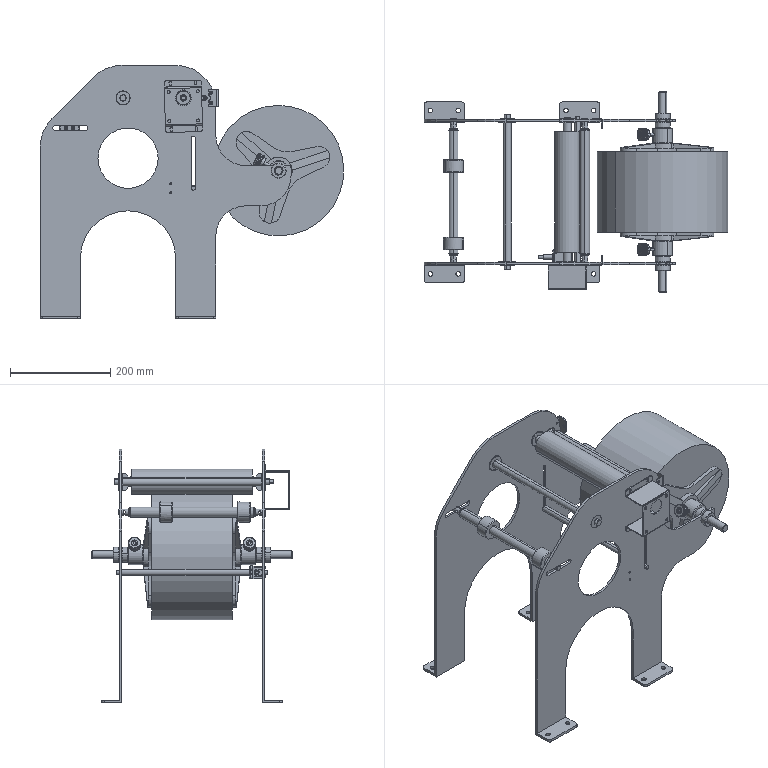Assembly | SolidWorks | mm | 29 component files | 32 solids | 1047 faces | box 605 x 400 x 505 mm | volume 10515334 mm3 | plane 504 | cylinder 399 | cone 100 | spline 44 | commonest cylinder face diameters 1 x52 10 x36 12 x31 16 x30 6 x26 5 x18 28 x16 4.2 x16
Bill of materials:
AdjustmentRing | 1 |  | Large-diameter cylindrical body with smaller coaxial stepped shaft ends at both ends; the ends are not symmetric, with more steps at one end.
AdjustmentRod | 1 |  | Long slender cylindrical shaft with a short reduced-diameter end step at each end.
F6001ZZ | 4 |  | Flanged bushing-like ring: a thin wide flange joined to a shorter-diameter cylindrical body, with a straight central through-bore.
FilmTensionPlate | 2 |  | Sheet-like L-shaped (90-degree bent) bracket. One leg has two round holes with a semicircular notch on the edge between them. The other leg has one smaller hole and a large rounded corner.
FloatingRod | 1 |  | Long, very slender cylindrical shaft with short reduced-diameter end steps at both ends; similar in form to unnamed part but thinner relative to its length.
LocatingRing | 4 |  | Short thick ring/collar with chamfered outer edges, a large central bore, and one small radial hole through the outer surface.
MaterialBarrel | 1 |  | Thick cylindrical spacer or sleeve with a relatively small concentric through-bore.
MaterialRod | 1 |  | Plain straight cylindrical rod/pin of constant diameter, with possible small chamfers at the ends.
MirrorVerticalPlate_Default_ByProcessing | 1 |  | Flat plate with an irregular outline, standing on two short bent-over foot tabs at the bottom of two legs separated by an arched opening. The plate has a large round hole, two smaller round holes, several elongated slots, tiny holes, and a side arm with a small edge notch.
MotorBracket | 1 |  | Formed hat/U-channel bracket: a flat central web joined to two parallel side walls, each ending in an outward-turned flange. The web has a large central round hole and four round holes near its corners. Each flange has two elongated slots.
NBM6_25_25_B_NBM6-25-25-B | 2 |  | Knob with a cylindrical head fluted around its edge, a smaller coaxial neck/collar, and a long smooth cylindrical shank. The head's end face has a recessed concentric ring feature.
Plug | 2 |  | Three-armed wing/star-shaped knob or handle plate with rounded arm tips, a central through-hole, and a raised conical/stepped hub boss on one face. The arms taper thinner toward their tips.
RetainingRing | 2 |  | Short thick-walled cylindrical sleeve/spacer with a plain through bore and small chamfers on the outer edges of both end faces.
SlideRod | 2 |  | Long slender cylindrical pin or shaft, symmetric end to end, with stepped reduced-diameter journals at both ends; each end journal has a small transverse cross hole, and there is a short shoulder/collar step between the main body and each journal.
TL_N5ME2 | 1 |  | Rectangular box-shaped body. A two-diameter stepped cylindrical shaft sticks out of one end face. Short cylindrical studs stick out of the side faces: two on one face and at least one on an adjacent face. The face opposite the shaft has a faint engraved circle with crosshair lines.
TopMaterialTray | 2 |  | Cylindrical sleeve/spacer with a through bore, chamfered outer end edges, a chamfered or countersunk bore entry, and one small radial cross hole near one end.
VerticalPlate_Default_ByProcessing | 1 |  | Thin flat sheet-metal-style bracket plate with an irregular outline. It has a large round hole, a tall arched cutout between two legs, several straight slots and small round holes, and a side tab ending in a hook-like notch. The bottom of each leg is bent 90 degrees into a foot tab with two small holes.
Mates:
1. concentric | MaterialRod-1 face at (155, -199.957, -145) dir (0, 1, 0) r 8 | TopMaterialTray-1 face at (155, 127, -145) dir (0, -1, 0) r 8
2. concentric | TopMaterialTray-1 face at (137.325, 114.5, -135.64) dir (-0.8837, 0, 0.468) r 2.5 | NBM6_25_25_B_NBM6-25-25-B-2 face at (147.93, 114.5, -141.256) dir (-0.8837, 0, 0.468) r 3
3. tangent | MaterialRod-1 face at (155, -199.957, -145) dir (0, 1, 0) r 8 | NBM6_25_25_B_NBM6-25-25-B-2 face at (146.871, 115.255, -143.257) dir (0.8837, 0, -0.468)
4. concentric | MaterialRod-1 face at (155, -199.957, -145) dir (0, 1, 0) r 8 | LocatingRing-3 face at (155, 128, -145) dir (0, 1, 0) r 8
5. coincident | LocatingRing-3 face at (155, 140, -145) dir (0, 1, 0) | VerticalPlate_Default_ByProcessing-3 face at (-145, 140, -185) dir (0, -1, 0)
6. concentric | MaterialRod-1 face at (155, -199.957, -145) dir (0, 1, 0) r 8 | LocatingRing-5 face at (155, 145, -145) dir (0, 1, 0) r 8
7. coincident | VerticalPlate_Default_ByProcessing-3 face at (-145, 145, -185) dir (0, 1, 0) | LocatingRing-5 face at (155, 145, -145) dir (0, -1, 0)
8. concentric | AdjustmentRing-2 face at (-35, 148, 0) dir (0, 1, 0) r 6 | F6001ZZ-3 face at (-35, 146, 0) dir (0, -1, 0) r 6
9. coincident | AdjustmentRing-2 face at (-36.452, 138, 5.822) dir (0, 1, 0) | F6001ZZ-3 face at (-35, 138, 0) dir (0, -1, 0)
10. concentric | MaterialRod-1 face at (155, -199.957, -145) dir (0, 1, 0) r 8 | MaterialBarrel-2 face at (155, 80, -145) dir (0, -1, 0) r 130
11. concentric | MaterialRod-1 face at (155, -199.957, -145) dir (0, 1, 0) r 8 | VerticalPlate_Default_ByProcessing-3 face at (155, 140, -145) dir (0, 1, 0) r 8
12. concentric | F6001ZZ-3 face at (-35, 138, 0) dir (0, 1, 0) r 14 | VerticalPlate_Default_ByProcessing-3 face at (-35, 140, 0) dir (0, 1, 0) r 14
13. coincident | F6001ZZ-3 face at (-35, 140, 0) dir (0, 1, 0) | VerticalPlate_Default_ByProcessing-3 face at (-145, 140, -185) dir (0, -1, 0)
14. slot | SlideRod-2 face at (0, 0, 0) dir (0, 1, 0) r 6 | VerticalPlate_Default_ByProcessing-3 face at (7.5, 140, -5) dir (0, 0, 1)
15. parallel | VerticalPlate_Default_ByProcessing-3 face at (7.5, 140, -5) dir (0, 0, 1) | SlideRod-2 face at (-15.013, 147, 5) dir (0, 0, 1)
16. coincident | VerticalPlate_Default_ByProcessing-3 face at (-145, 145, -185) dir (0, 1, 0) | FilmTensionPlate-1 face at (34.5, 145, 0) dir (0, -1, 0)
17. concentric | VerticalPlate_Default_ByProcessing-3 face at (20, 145, 10) dir (0, 1, 0) r 2.1 | FilmTensionPlate-1 face at (20, 145, 10) dir (0, 1, 0) r 3.25
18. concentric | VerticalPlate_Default_ByProcessing-3 face at (20, 145, -10) dir (0, 1, 0) r 2.1 | FilmTensionPlate-1 face at (20, 145, -10) dir (0, 1, 0) r 3.25
19. coincident | VerticalPlate_Default_ByProcessing-3 face at (-145, 140, -185) dir (0, -1, 0) | SlideRod-2 face at (0, 140, 0) dir (0, 1, 0)
20. slot | VerticalPlate_Default_ByProcessing-3 face at (-19, 140, -80) dir (1, 0, 0) | FloatingRod-1 face at (-15, 0, -180) dir (0, -1, 0) r 4
21. width | FloatingRod-1 face at (-15, 150, -180) dir (0, 1, 0) | FloatingRod-1 face at (-15, -150, -180) dir (0, -1, 0) | VerticalPlate_Default_ByProcessing-3 face at (-145, 145, -185) dir (0, 1, 0) | MirrorVerticalPlate_Default_ByProcessing-5 face at (-145, -145, -185) dir (0, -1, 0)
22. coincident | MirrorVerticalPlate_Default_ByProcessing-5 face at (-145, -145, -185) dir (0, -1, 0) | MotorBracket-1 face at (-34.647, -145, -16.496) dir (0, 1, 0)
23. concentric | AdjustmentRing-2 face at (-35, 148, 0) dir (0, 1, 0) r 4 | MotorBracket-1 face at (-35, -193, 0) dir (0, -1, 0) r 16
24. coincident | TL_N5ME2-1 face at (-56.223, -140, -167.712) dir (0, -1, 0) | MirrorVerticalPlate_Default_ByProcessing-5 face at (-145, -140, -185) dir (0, 1, 0)
25. coincident | VerticalPlate_Default_ByProcessing-3 face at (-230, 140, -65) dir (0, 0, 1) | SlideRod-3 face at (-276.717, 147, -65) dir (0, 0, -1)
26. coincident | SlideRod-2 face at (0, 147, 0) dir (0, 1, 0) | SlideRod-3 face at (-261.704, 147, -60) dir (0, 1, 0)
27. concentric | VerticalPlate_Default_ByProcessing-3 face at (-155, 140, 0) dir (0, 1, 0) r 14 | F6001ZZ-10 face at (-155, 138, 0) dir (0, 1, 0) r 14
28. coincident | VerticalPlate_Default_ByProcessing-3 face at (-145, 140, -185) dir (0, -1, 0) | F6001ZZ-10 face at (-155, 140, 0) dir (0, 1, 0)
29. concentric | SlideRod-3 face at (-261.704, 0, -60) dir (0, 1, 0) r 10 | RetainingRing-3 face at (-261.704, 64.098, -60) dir (0, -1, 0) r 8
30. concentric | SlideRod-3 face at (-261.704, 0, -60) dir (0, 1, 0) r 10 | RetainingRing-4 face at (-261.704, -90.627, -60) dir (0, -1, 0) r 8
31. concentric | F6001ZZ-10 face at (-155, 146, 0) dir (0, -1, 0) r 6 | AdjustmentRod-2 face at (-155, 0, 0) dir (0, -1, 0) r 6
32. coincident | F6001ZZ-10 face at (-155, 138, 0) dir (0, -1, 0) | AdjustmentRod-2 face at (-149.252, 138, 1.72) dir (0, 1, 0)
33. concentric | MaterialRod-1 face at (155, -199.957, -145) dir (0, 1, 0) r 8 | Plug-2 face at (155, 97, -145) dir (0, -1, 0) r 12.5
34. coincident | MaterialBarrel-2 face at (155, 80, -145) dir (0, 1, 0) | Plug-2 face at (155, 80, -145) dir (0, -1, 0)
35. coincident | TopMaterialTray-1 face at (155, 97, -145) dir (0, -1, 0) | Plug-2 face at (155, 97, -145) dir (0, 1, 0)
36. width | VerticalPlate_Default_ByProcessing-3 face at (-145, 145, -185) dir (0, 1, 0) | MirrorVerticalPlate_Default_ByProcessing-5 face at (-145, -145, -185) dir (0, -1, 0) | MaterialBarrel-2 face at (155, -80, -145) dir (0, -1, 0) | MaterialBarrel-2 face at (155, 80, -145) dir (0, 1, 0)